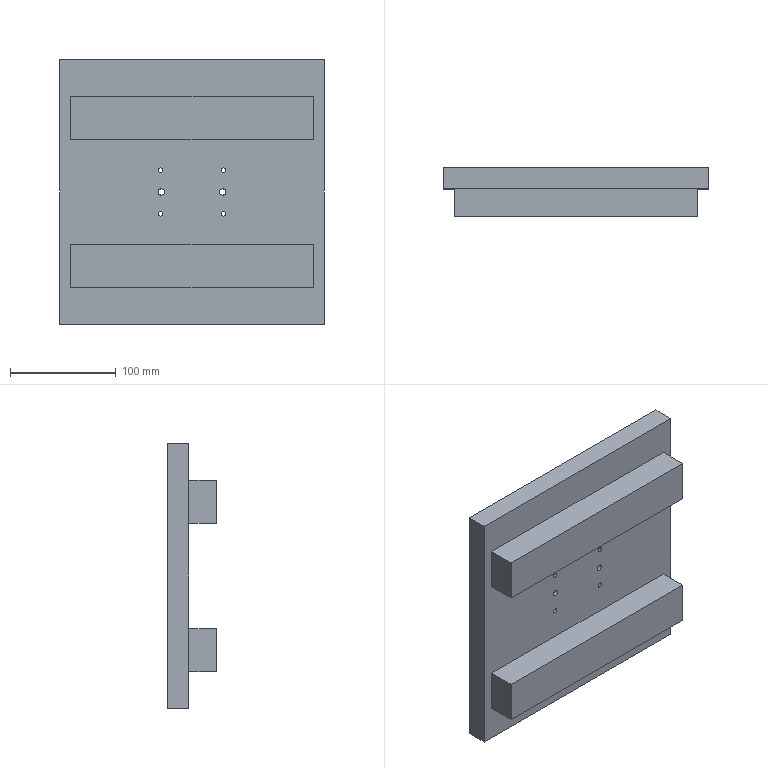Component | SolidWorks | WorkPlatform-1 | 1 solid | 43 faces | box 250 x 46 x 250 mm | volume 1732663 mm3 | cylinder 22 | plane 21 | commonest cylinder face diameters 4.542 x8 8.034 x8 5.965 x4 18.759 x2
build123d program:
from build123d import *

# Parameters (mm, degrees)
SKETCH1_W           = 230
SKETCH1_H           = 230
BOSS_EXTRUDE1_DEPTH = 20
SKETCH3_R           = 4.017
CUT_EXTRUDE1_DEPTH  = 10
SKETCH4_R           = 2.271
CUT_EXTRUDE2_DEPTH  = 48
SKETCH5_R           = 2.983
CUT_EXTRUDE3_DEPTH  = 29
SKETCH6_W           = 40.761
SKETCH6_H           = 230
BOSS_EXTRUDE2_DEPTH = 26.003
SKETCH7_R           = 8.316
CUT_EXTRUDE4_DEPTH  = 1.5
SKETCH8_W           = 250
SKETCH8_H           = 250
SKETCH8_W_2         = 230
SKETCH8_H_2         = 230
BOSS_EXTRUDE3_DEPTH = 20
BOSS_EXTRUDE4_START = 1.5
SKETCH9_R           = 8.316
BOSS_EXTRUDE4_DEPTH = 1.5
SKETCH10_R          = 9.38
CUT_EXTRUDE5_DEPTH  = 4


with BuildPart() as part:
    # Sketch1 → Boss-Extrude1 (new body)
    with BuildSketch(Plane(origin=(0, 0, 0), x_dir=(1, 0, 0), z_dir=(0, 1, 0))):
        Rectangle(SKETCH1_W, SKETCH1_H)
    extrude(amount=BOSS_EXTRUDE1_DEPTH)

    # Sketch3 → Cut-Extrude1 (cut)
    with BuildSketch(Plane(origin=(0, 20, 0), x_dir=(1, 0, 0), z_dir=(0, 1, 0))):
        with Locations(Location((20.473, 29.799, 0), (0, 0, 270))):
            Circle(SKETCH3_R)
        with Locations(Location((20.473, -29.799, 0), (0, 0, 90))):
            Circle(SKETCH3_R)
        with Locations(Location((-20.473, -29.799, 0), (0, 0, 270))):
            Circle(SKETCH3_R)
        with Locations(Location((-20.473, 29.799, 0), (0, 0, 90))):
            Circle(SKETCH3_R)
    extrude(amount=-CUT_EXTRUDE1_DEPTH, mode=Mode.SUBTRACT)

    # Sketch4 → Cut-Extrude2 (cut)
    with BuildSketch(Plane(origin=(0, 10, 0), x_dir=(1, 0, 0), z_dir=(0, 1, 0))):
        with Locations(Location((20.473, 29.799, 0), (0, 0, 270))):
            Circle(SKETCH4_R)
        with Locations(Location((20.473, -29.799, 0), (0, 0, 270))):
            Circle(SKETCH4_R)
        with Locations(Location((-20.473, -29.799, 0), (0, 0, 270))):
            Circle(SKETCH4_R)
        with Locations(Location((-20.473, 29.799, 0), (0, 0, 270))):
            Circle(SKETCH4_R)
    extrude(amount=-CUT_EXTRUDE2_DEPTH, mode=Mode.SUBTRACT)

    # Sketch5 → Cut-Extrude3 (cut)
    with BuildSketch(Plane(origin=(0, 20, 0), x_dir=(1, 0, 0), z_dir=(0, 1, 0))):
        with Locations(Location((0, 29.142, 0), (0, 0, 270))):
            Circle(SKETCH5_R)
        with Locations(Location((0, -29.142, 0), (0, 0, 270))):
            Circle(SKETCH5_R)
    extrude(amount=-CUT_EXTRUDE3_DEPTH, mode=Mode.SUBTRACT)

    # Sketch6 → Boss-Extrude2 (add)
    with BuildSketch(Plane.XZ):
        with Locations((-70.515, 0)):
            Rectangle(SKETCH6_W, SKETCH6_H)
    boss_extrude2 = extrude(amount=BOSS_EXTRUDE2_DEPTH)

    # Mirror1: Boss-Extrude2 across plane
    add(boss_extrude2.mirror(Plane.ZY))

    # Sketch7 → Cut-Extrude4 (cut)
    with BuildSketch(Plane.XY.offset(115)):
        with Locations((67.772, -0.5408)):
            Circle(SKETCH7_R)
    extrude(amount=-CUT_EXTRUDE4_DEPTH, mode=Mode.SUBTRACT)

    # Sketch8 → Boss-Extrude3 (add)
    with BuildSketch(Plane(origin=(0, 20, 0), x_dir=(1, 0, 0), z_dir=(0, 1, 0))):
        Rectangle(SKETCH8_W, SKETCH8_H)
        Rectangle(SKETCH8_W_2, SKETCH8_H_2, mode=Mode.SUBTRACT)
    extrude(amount=-BOSS_EXTRUDE3_DEPTH)

    # Sketch9 → Boss-Extrude4 (add)
    with BuildSketch(Plane.XY.offset(113.5).offset(BOSS_EXTRUDE4_START)):
        with Locations((67.772, -0.5408)):
            Circle(SKETCH9_R)
    extrude(amount=-BOSS_EXTRUDE4_DEPTH)

    # Sketch10 → Cut-Extrude5 (cut)
    with BuildSketch(Plane.XY.offset(115)):
        with Locations((69.517, -12.625)):
            Circle(SKETCH10_R)
    extrude(amount=-CUT_EXTRUDE5_DEPTH, mode=Mode.SUBTRACT)


solid = part.part

# Placed as in the assembly
solid = solid.moved(Location((56.772, 96.74, 0), (0, 90, 0)))